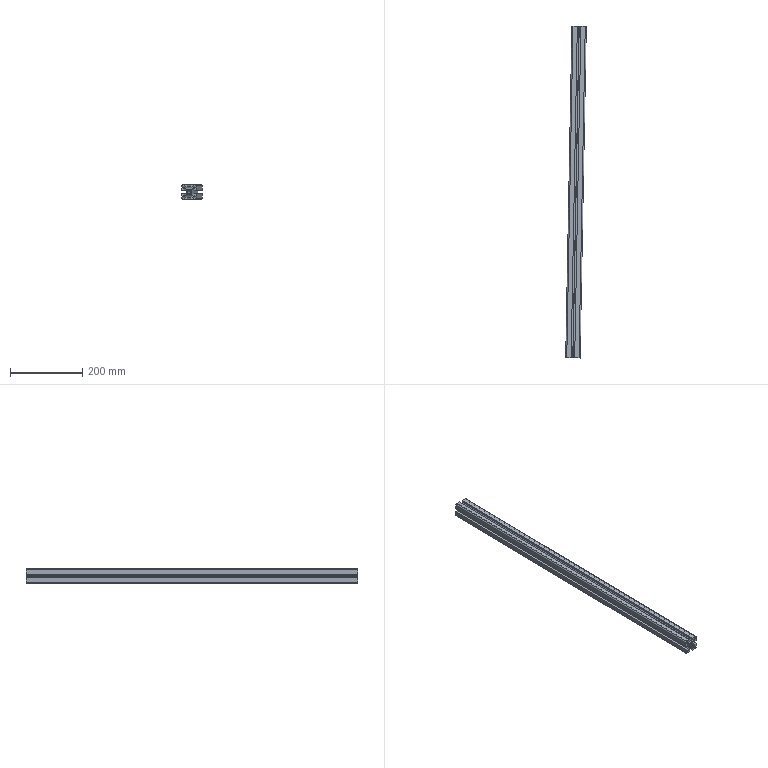Component | SolidWorks | A6061-4040-L920_AluminumExtrusion-1 | 1 solid | 111 faces | volume 572286 mm3 | plane 74 | cylinder 37 | commonest cylinder face diameters 2 x28 10.5 x5 6 x4 | material 6061 Alloy